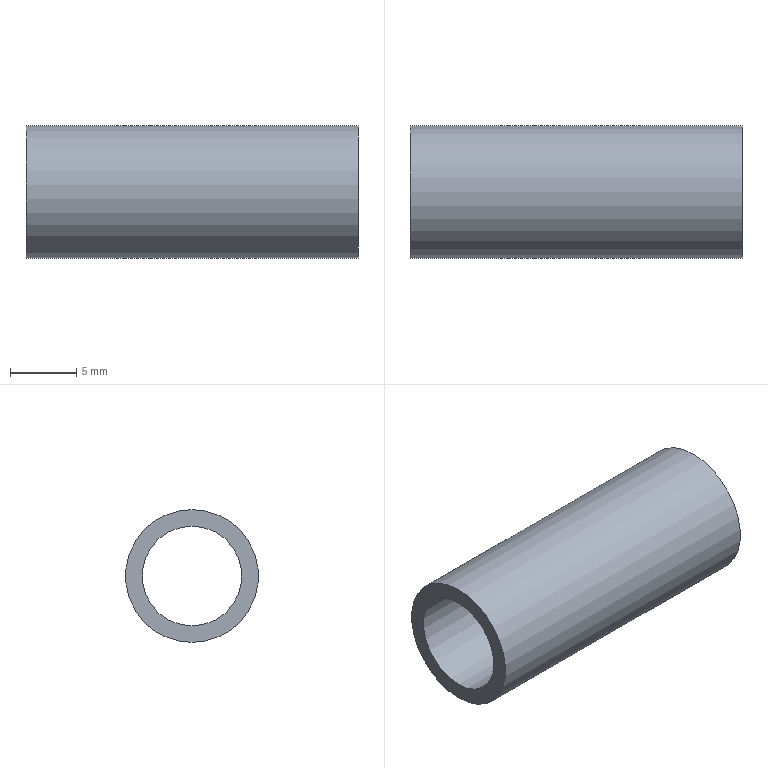Component | NX | VENT_PIPE | 1 solid | 4 faces | box 25 x 10 x 10 mm | volume 859 mm3 | cylinder 2 | plane 2 | commonest cylinder face diameters 10 x1 7.5 x1
STEP:
#1=CARTESIAN_POINT('',(0.,0.,0.));
#2=DIRECTION('',(0.,0.,1.));
#3=DIRECTION('',(1.,0.,0.));
#4=AXIS2_PLACEMENT_3D('',#1,#2,#3);
#5=CARTESIAN_POINT('',(-161.,-59.,23.5));
#6=VERTEX_POINT('',#5);
#7=CARTESIAN_POINT('',(-161.,-59.,18.5));
#8=DIRECTION('',(1.,0.,0.));
#9=DIRECTION('',(0.,0.,1.));
#10=AXIS2_PLACEMENT_3D('',#7,#8,#9);
#11=CIRCLE('',#10,5.);
#12=CARTESIAN_POINT('',(-161.,-59.,18.5));
#13=DIRECTION('',(1.,0.,0.));
#14=DIRECTION('',(0.,0.,-1.));
#15=AXIS2_PLACEMENT_3D('',#12,#13,#14);
#16=CYLINDRICAL_SURFACE('',#15,5.);
#17=CARTESIAN_POINT('',(3.142,0.));
#18=DIRECTION('',(1.,0.));
#19=VECTOR('',#18,1.);
#20=LINE('',#17,#19);
#21=(GEOMETRIC_REPRESENTATION_CONTEXT(2)PARAMETRIC_REPRESENTATION_CONTEXT()REPRESENTATION_CONTEXT('',''));
#22=DEFINITIONAL_REPRESENTATION('',(#20),#21);
#23=PCURVE('',#16,#22);
#24=CARTESIAN_POINT('',(-161.,-59.,18.5));
#25=DIRECTION('',(1.,0.,0.));
#26=DIRECTION('',(0.,0.,-1.));
#27=AXIS2_PLACEMENT_3D('',#24,#25,#26);
#28=PLANE('',#27);
#29=CARTESIAN_POINT('',(0.,0.));
#30=DIRECTION('',(-1.,0.));
#31=AXIS2_PLACEMENT_2D('',#29,#30);
#32=CIRCLE('',#31,5.);
#33=(GEOMETRIC_REPRESENTATION_CONTEXT(2)PARAMETRIC_REPRESENTATION_CONTEXT()REPRESENTATION_CONTEXT('',''));
#34=DEFINITIONAL_REPRESENTATION('',(#32),#33);
#35=PCURVE('',#28,#34);
#36=SURFACE_CURVE('',#11,(#23,#35),.PCURVE_S1.);
#37=EDGE_CURVE('',#6,#6,#36,.T.);
#38=ORIENTED_EDGE('',*,*,#37,.T.);
#39=CARTESIAN_POINT('',(-136.,-59.,23.5));
#40=VERTEX_POINT('',#39);
#41=CARTESIAN_POINT('',(-161.,-59.,23.5));
#42=CARTESIAN_POINT('',(-136.,-59.,23.5));
#43=B_SPLINE_CURVE_WITH_KNOTS('',1,(#41,#42),.UNSPECIFIED.,.F.,.F.,(2,2),(0.,25.),.PIECEWISE_BEZIER_KNOTS.);
#44=CARTESIAN_POINT('',(9.425,0.));
#45=DIRECTION('',(0.,1.));
#46=VECTOR('',#45,1.);
#47=LINE('',#44,#46);
#48=(GEOMETRIC_REPRESENTATION_CONTEXT(2)PARAMETRIC_REPRESENTATION_CONTEXT()REPRESENTATION_CONTEXT('',''));
#49=DEFINITIONAL_REPRESENTATION('',(#47),#48);
#50=PCURVE('',#16,#49);
#51=CARTESIAN_POINT('',(3.142,0.));
#52=DIRECTION('',(0.,1.));
#53=VECTOR('',#52,1.);
#54=LINE('',#51,#53);
#55=(GEOMETRIC_REPRESENTATION_CONTEXT(2)PARAMETRIC_REPRESENTATION_CONTEXT()REPRESENTATION_CONTEXT('',''));
#56=DEFINITIONAL_REPRESENTATION('',(#54),#55);
#57=PCURVE('',#16,#56);
#58=SEAM_CURVE('',#43,(#50,#57),.PCURVE_S1.);
#59=EDGE_CURVE('',#6,#40,#58,.T.);
#60=ORIENTED_EDGE('',*,*,#59,.T.);
#61=CARTESIAN_POINT('',(-136.,-59.,18.5));
#62=DIRECTION('',(1.,0.,0.));
#63=DIRECTION('',(0.,0.,1.));
#64=AXIS2_PLACEMENT_3D('',#61,#62,#63);
#65=CIRCLE('',#64,5.);
#66=CARTESIAN_POINT('',(3.142,25.));
#67=DIRECTION('',(1.,0.));
#68=VECTOR('',#67,1.);
#69=LINE('',#66,#68);
#70=(GEOMETRIC_REPRESENTATION_CONTEXT(2)PARAMETRIC_REPRESENTATION_CONTEXT()REPRESENTATION_CONTEXT('',''));
#71=DEFINITIONAL_REPRESENTATION('',(#69),#70);
#72=PCURVE('',#16,#71);
#73=CARTESIAN_POINT('',(-136.,-59.,18.5));
#74=DIRECTION('',(1.,0.,0.));
#75=DIRECTION('',(0.,0.,-1.));
#76=AXIS2_PLACEMENT_3D('',#73,#74,#75);
#77=PLANE('',#76);
#78=CARTESIAN_POINT('',(0.,0.));
#79=DIRECTION('',(-1.,0.));
#80=AXIS2_PLACEMENT_2D('',#78,#79);
#81=CIRCLE('',#80,5.);
#82=(GEOMETRIC_REPRESENTATION_CONTEXT(2)PARAMETRIC_REPRESENTATION_CONTEXT()REPRESENTATION_CONTEXT('',''));
#83=DEFINITIONAL_REPRESENTATION('',(#81),#82);
#84=PCURVE('',#77,#83);
#85=SURFACE_CURVE('',#65,(#72,#84),.PCURVE_S1.);
#86=EDGE_CURVE('',#40,#40,#85,.T.);
#87=ORIENTED_EDGE('',*,*,#86,.F.);
#88=ORIENTED_EDGE('',*,*,#59,.F.);
#89=EDGE_LOOP('',(#38,#60,#87,#88));
#90=FACE_BOUND('',#89,.T.);
#91=ADVANCED_FACE('',(#90),#16,.T.);
#92=CARTESIAN_POINT('',(-161.,-59.,22.25));
#93=VERTEX_POINT('',#92);
#94=CARTESIAN_POINT('',(-161.,-59.,18.5));
#95=DIRECTION('',(1.,0.,0.));
#96=DIRECTION('',(0.,0.,1.));
#97=AXIS2_PLACEMENT_3D('',#94,#95,#96);
#98=CIRCLE('',#97,3.75);
#99=CARTESIAN_POINT('',(-161.,-59.,18.5));
#100=DIRECTION('',(1.,0.,0.));
#101=DIRECTION('',(0.,0.,-1.));
#102=AXIS2_PLACEMENT_3D('',#99,#100,#101);
#103=CYLINDRICAL_SURFACE('',#102,3.75);
#104=CARTESIAN_POINT('',(3.142,0.));
#105=DIRECTION('',(1.,0.));
#106=VECTOR('',#105,1.);
#107=LINE('',#104,#106);
#108=(GEOMETRIC_REPRESENTATION_CONTEXT(2)PARAMETRIC_REPRESENTATION_CONTEXT()REPRESENTATION_CONTEXT('',''));
#109=DEFINITIONAL_REPRESENTATION('',(#107),#108);
#110=PCURVE('',#103,#109);
#111=CARTESIAN_POINT('',(0.,0.));
#112=DIRECTION('',(-1.,0.));
#113=AXIS2_PLACEMENT_2D('',#111,#112);
#114=CIRCLE('',#113,3.75);
#115=(GEOMETRIC_REPRESENTATION_CONTEXT(2)PARAMETRIC_REPRESENTATION_CONTEXT()REPRESENTATION_CONTEXT('',''));
#116=DEFINITIONAL_REPRESENTATION('',(#114),#115);
#117=PCURVE('',#28,#116);
#118=SURFACE_CURVE('',#98,(#110,#117),.PCURVE_S1.);
#119=EDGE_CURVE('',#93,#93,#118,.T.);
#120=ORIENTED_EDGE('',*,*,#119,.T.);
#121=CARTESIAN_POINT('',(-136.,-59.,22.25));
#122=VERTEX_POINT('',#121);
#123=CARTESIAN_POINT('',(-161.,-59.,22.25));
#124=CARTESIAN_POINT('',(-136.,-59.,22.25));
#125=B_SPLINE_CURVE_WITH_KNOTS('',1,(#123,#124),.UNSPECIFIED.,.F.,.F.,(2,2),(0.,25.),.PIECEWISE_BEZIER_KNOTS.);
#126=CARTESIAN_POINT('',(9.425,0.));
#127=DIRECTION('',(0.,1.));
#128=VECTOR('',#127,1.);
#129=LINE('',#126,#128);
#130=(GEOMETRIC_REPRESENTATION_CONTEXT(2)PARAMETRIC_REPRESENTATION_CONTEXT()REPRESENTATION_CONTEXT('',''));
#131=DEFINITIONAL_REPRESENTATION('',(#129),#130);
#132=PCURVE('',#103,#131);
#133=CARTESIAN_POINT('',(3.142,0.));
#134=DIRECTION('',(0.,1.));
#135=VECTOR('',#134,1.);
#136=LINE('',#133,#135);
#137=(GEOMETRIC_REPRESENTATION_CONTEXT(2)PARAMETRIC_REPRESENTATION_CONTEXT()REPRESENTATION_CONTEXT('',''));
#138=DEFINITIONAL_REPRESENTATION('',(#136),#137);
#139=PCURVE('',#103,#138);
#140=SEAM_CURVE('',#125,(#132,#139),.PCURVE_S1.);
#141=EDGE_CURVE('',#93,#122,#140,.T.);
#142=ORIENTED_EDGE('',*,*,#141,.T.);
#143=CARTESIAN_POINT('',(-136.,-59.,18.5));
#144=DIRECTION('',(1.,0.,0.));
#145=DIRECTION('',(0.,0.,1.));
#146=AXIS2_PLACEMENT_3D('',#143,#144,#145);
#147=CIRCLE('',#146,3.75);
#148=CARTESIAN_POINT('',(3.142,25.));
#149=DIRECTION('',(1.,0.));
#150=VECTOR('',#149,1.);
#151=LINE('',#148,#150);
#152=(GEOMETRIC_REPRESENTATION_CONTEXT(2)PARAMETRIC_REPRESENTATION_CONTEXT()REPRESENTATION_CONTEXT('',''));
#153=DEFINITIONAL_REPRESENTATION('',(#151),#152);
#154=PCURVE('',#103,#153);
#155=CARTESIAN_POINT('',(0.,0.));
#156=DIRECTION('',(-1.,0.));
#157=AXIS2_PLACEMENT_2D('',#155,#156);
#158=CIRCLE('',#157,3.75);
#159=(GEOMETRIC_REPRESENTATION_CONTEXT(2)PARAMETRIC_REPRESENTATION_CONTEXT()REPRESENTATION_CONTEXT('',''));
#160=DEFINITIONAL_REPRESENTATION('',(#158),#159);
#161=PCURVE('',#77,#160);
#162=SURFACE_CURVE('',#147,(#154,#161),.PCURVE_S1.);
#163=EDGE_CURVE('',#122,#122,#162,.T.);
#164=ORIENTED_EDGE('',*,*,#163,.F.);
#165=ORIENTED_EDGE('',*,*,#141,.F.);
#166=EDGE_LOOP('',(#120,#142,#164,#165));
#167=FACE_BOUND('',#166,.F.);
#168=ADVANCED_FACE('',(#167),#103,.F.);
#169=ORIENTED_EDGE('',*,*,#37,.F.);
#170=EDGE_LOOP('',(#169));
#171=FACE_BOUND('',#170,.T.);
#172=ORIENTED_EDGE('',*,*,#119,.T.);
#173=EDGE_LOOP('',(#172));
#174=FACE_BOUND('',#173,.T.);
#175=ADVANCED_FACE('',(#171,#174),#28,.F.);
#176=ORIENTED_EDGE('',*,*,#86,.T.);
#177=EDGE_LOOP('',(#176));
#178=FACE_BOUND('',#177,.T.);
#179=ORIENTED_EDGE('',*,*,#163,.F.);
#180=EDGE_LOOP('',(#179));
#181=FACE_BOUND('',#180,.T.);
#182=ADVANCED_FACE('',(#178,#181),#77,.T.);
#183=CLOSED_SHELL('',(#91,#168,#175,#182));
#184=MANIFOLD_SOLID_BREP('',#183);
#185=(LENGTH_UNIT()NAMED_UNIT(*)SI_UNIT(.MILLI.,.METRE.));
#186=UNCERTAINTY_MEASURE_WITH_UNIT(LENGTH_MEASURE(0.00001),#185,'','');
#187=(NAMED_UNIT(*)PLANE_ANGLE_UNIT()SI_UNIT($,.RADIAN.));
#188=(NAMED_UNIT(*)SI_UNIT($,.STERADIAN.)SOLID_ANGLE_UNIT());
#189=(GEOMETRIC_REPRESENTATION_CONTEXT(3)GLOBAL_UNCERTAINTY_ASSIGNED_CONTEXT((#186))GLOBAL_UNIT_ASSIGNED_CONTEXT((#185,#187,#188))REPRESENTATION_CONTEXT('',''));
#190=ADVANCED_BREP_SHAPE_REPRESENTATION('',(#4,#184),#189);